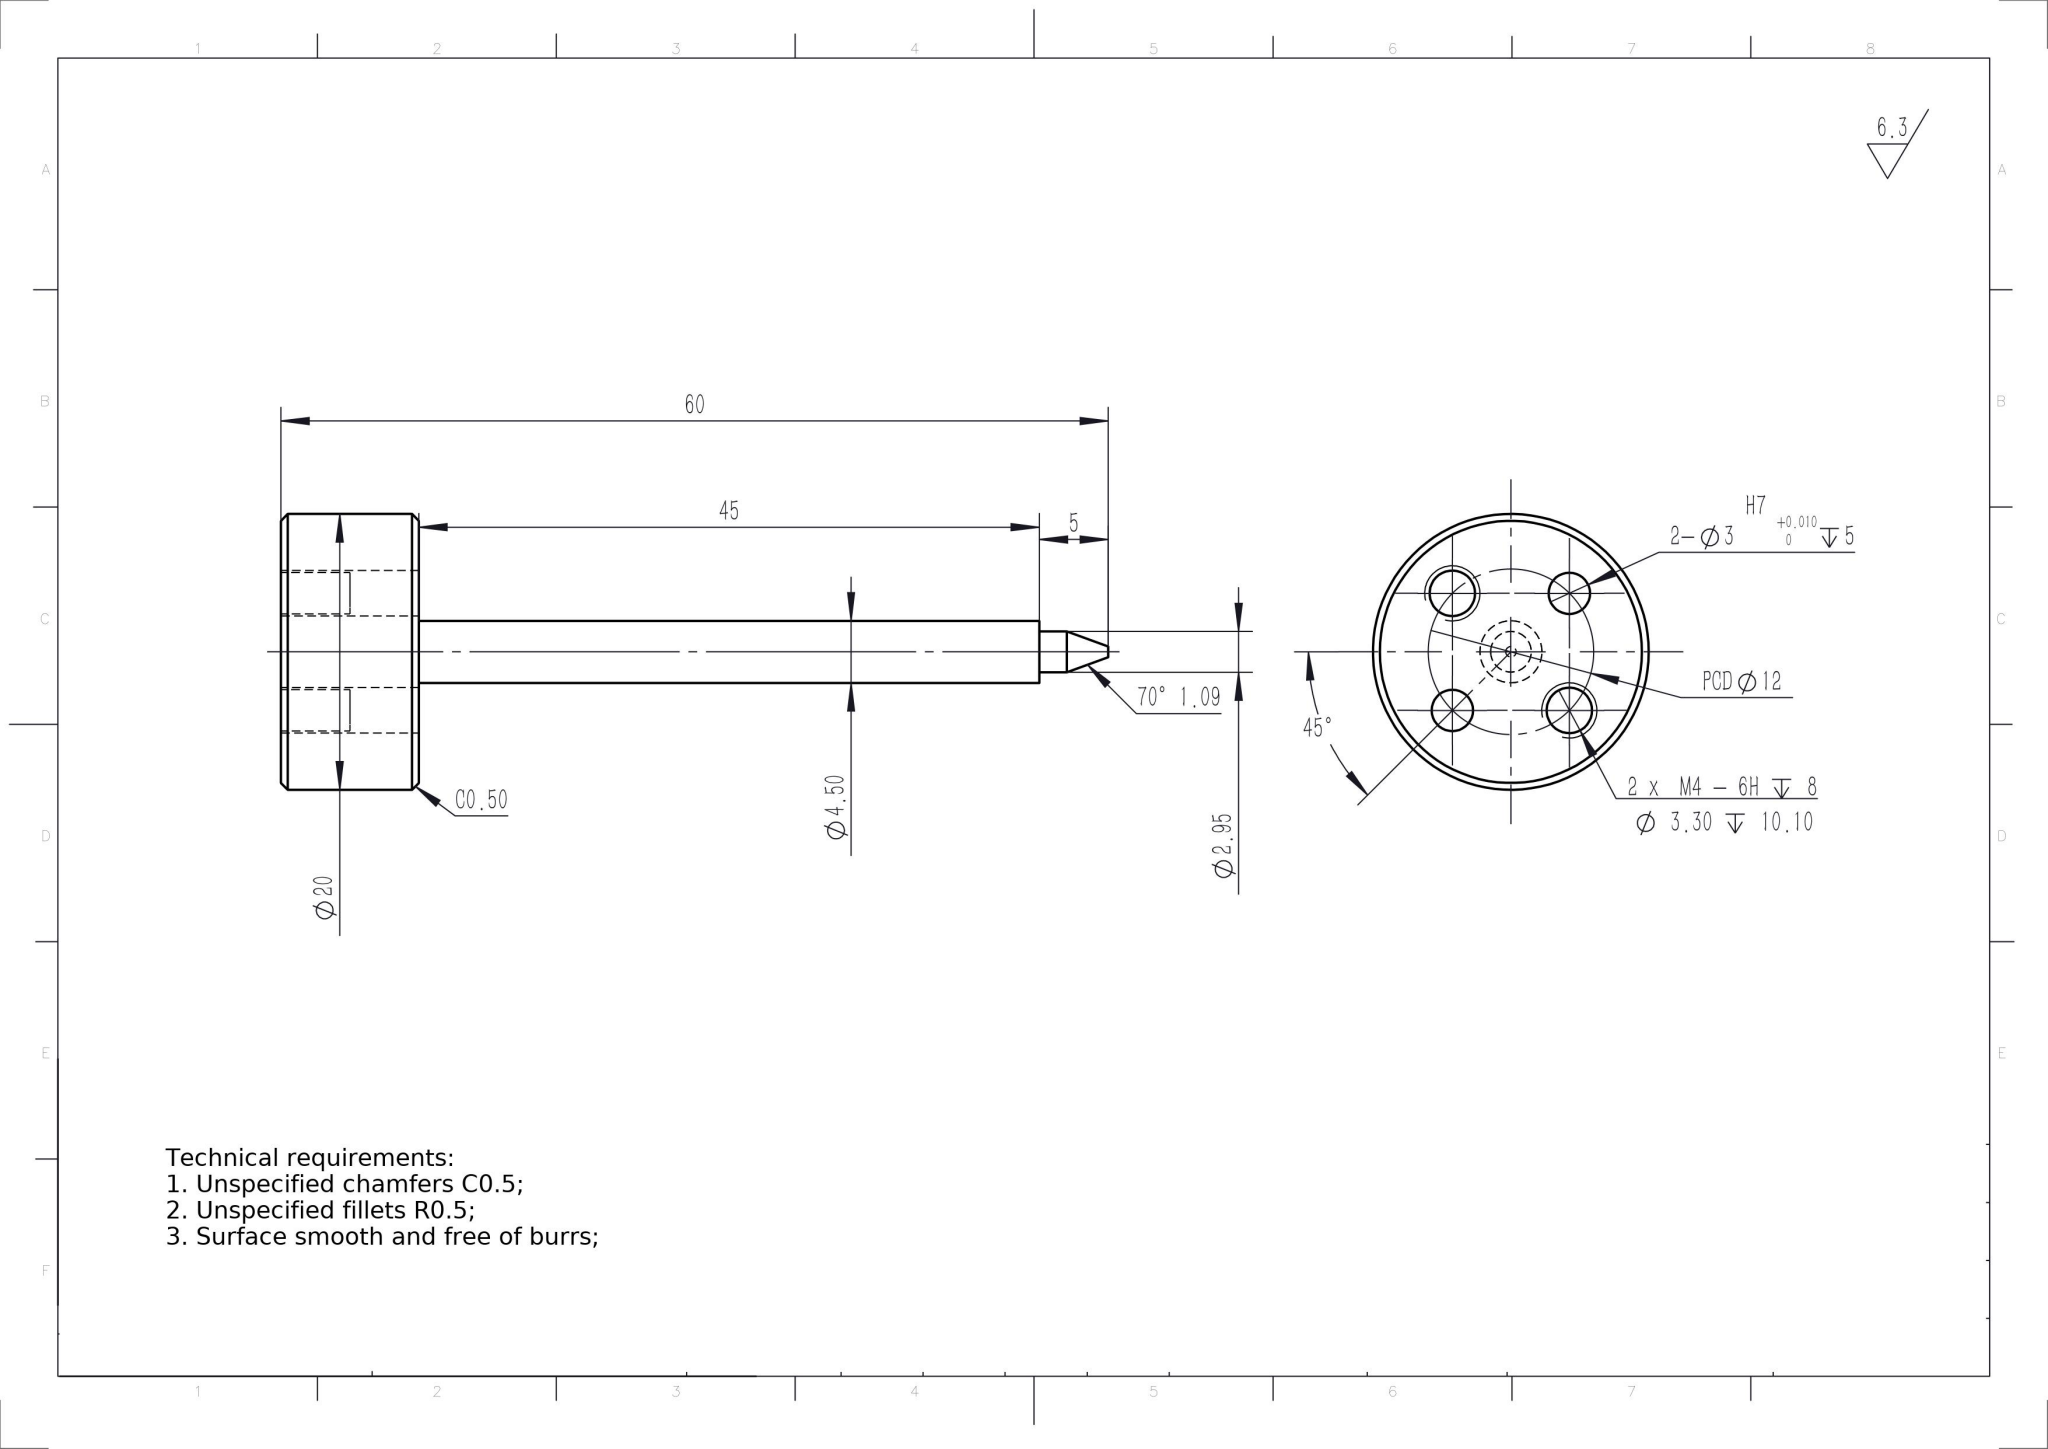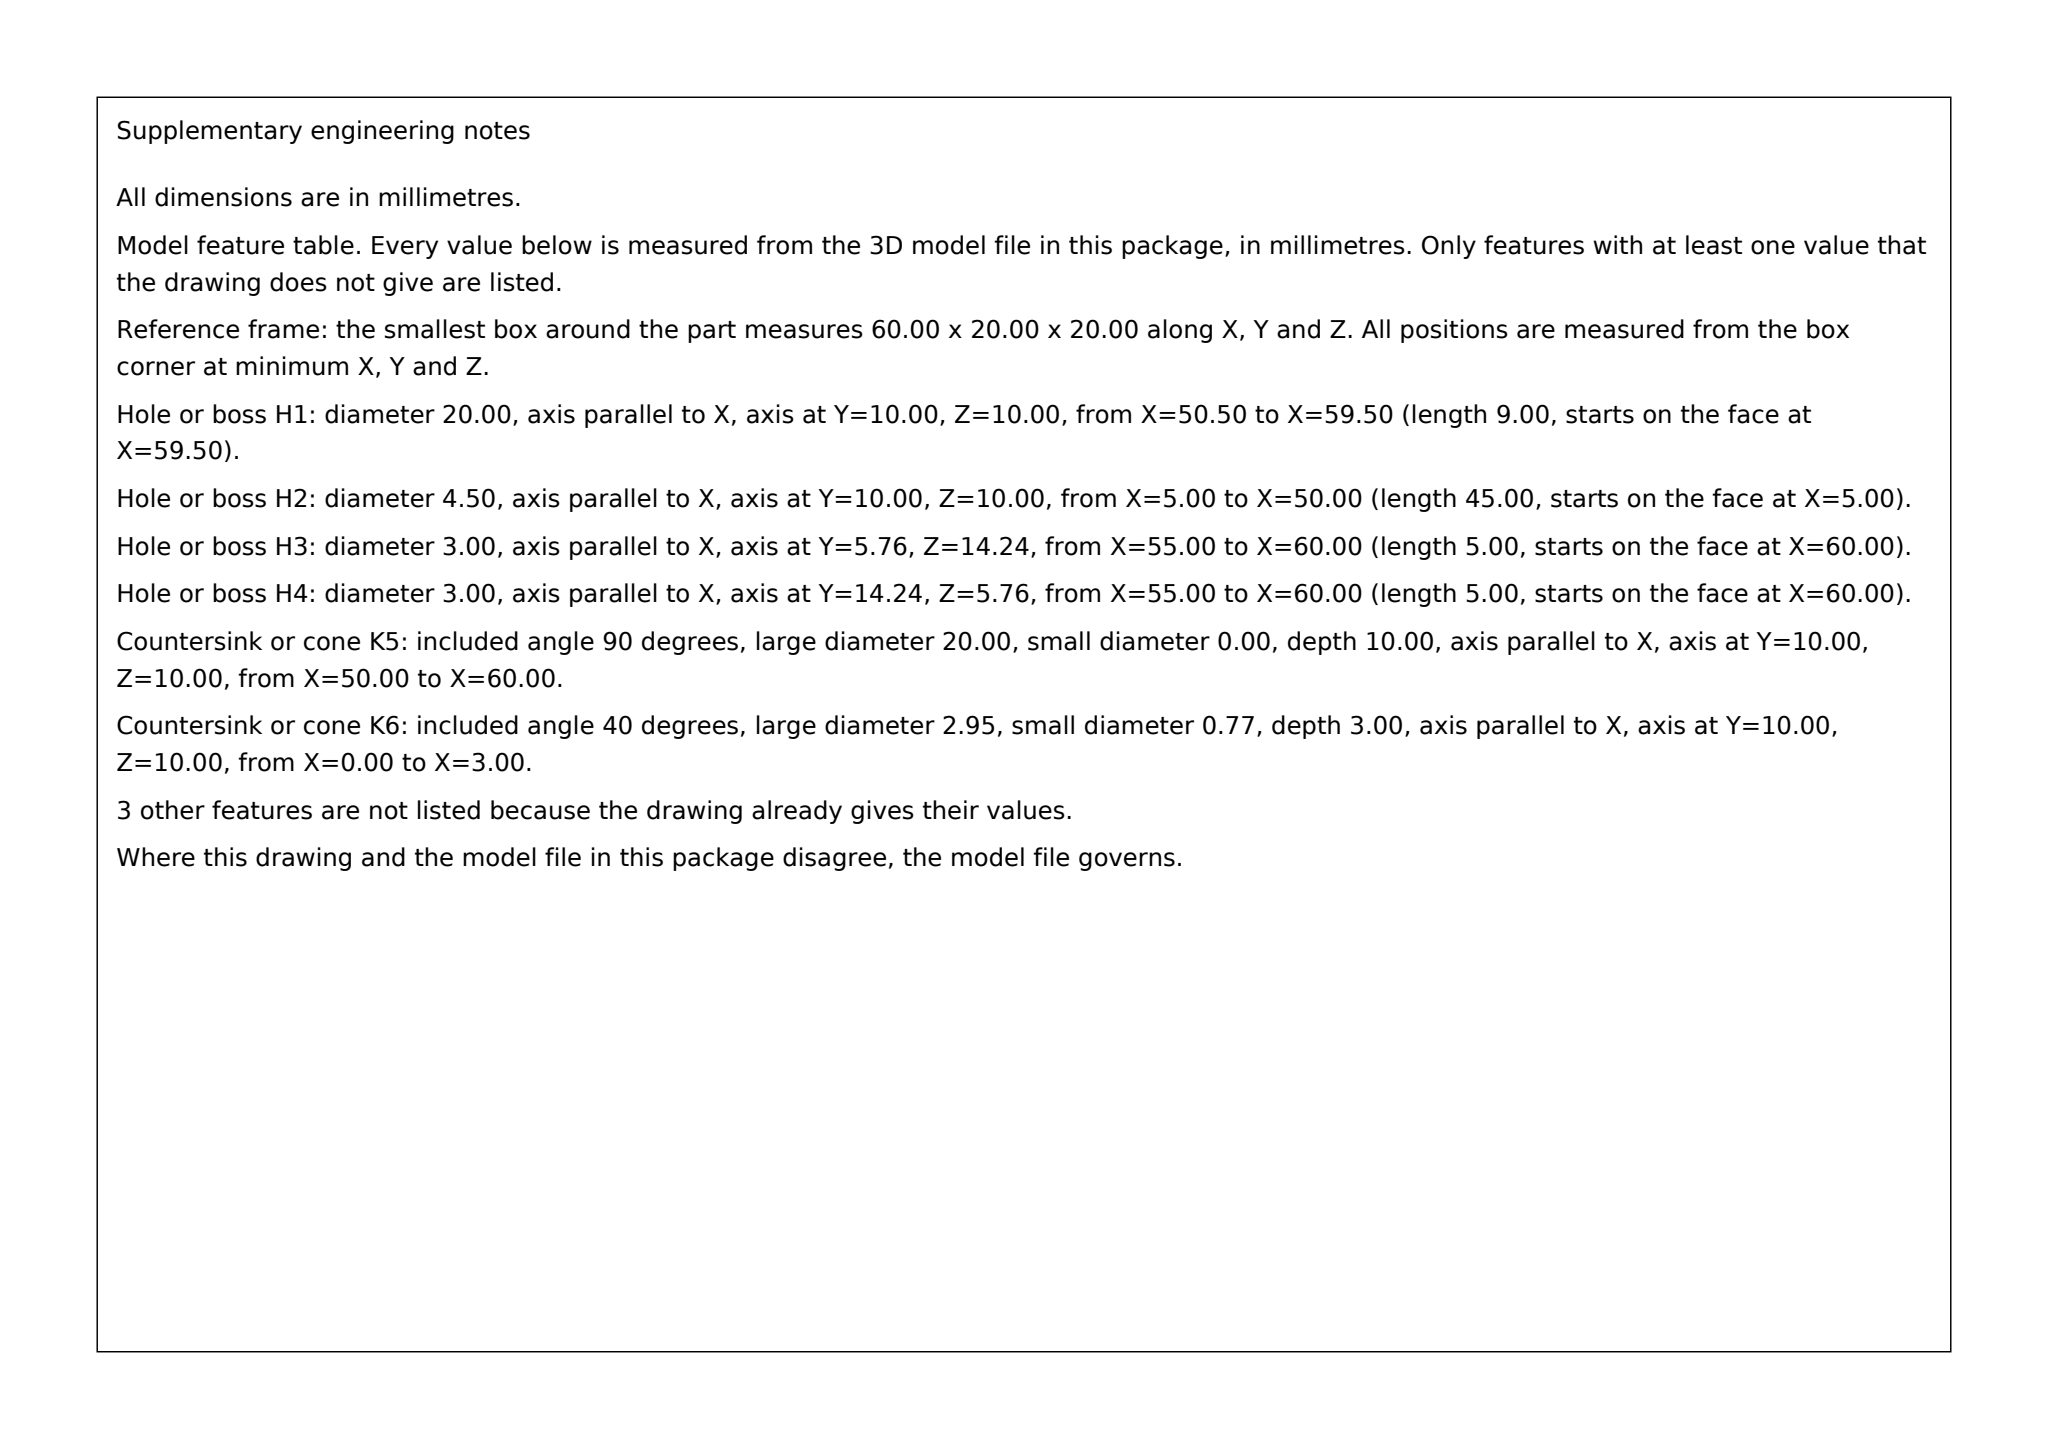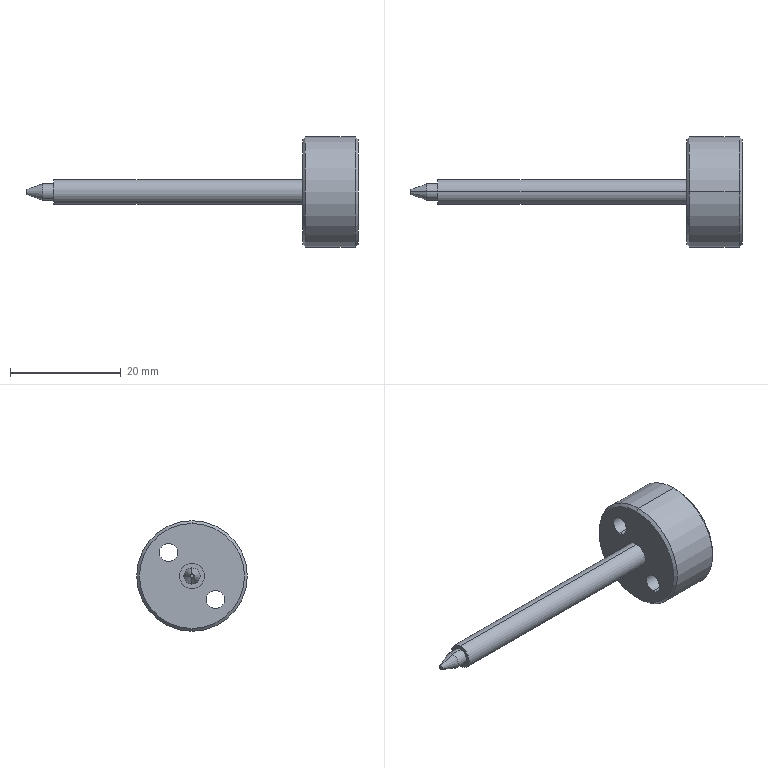Part | SolidWorks | mm | 1 solid | 26 faces | box 60 x 20 x 20 mm | volume 3623 mm3 | cylinder 14 | cone 6 | plane 6 | commonest cylinder face diameters 3.3 x4 3 x4 2.95 x2 20 x2 4.5 x2
build123d program:
from build123d import *

# Parameters (mm, degrees)
SKETCH1_R             = 2.25
BOSS_EXTRUDE1_DEPTH   = 45
SKETCH4_R             = 10
BOSS_EXTRUDE2_DEPTH   = 10
SKETCH6_R             = 2.5
CUT_EXTRUDE4_DEPTH    = 5
CHAMFER2_SIZE         = 0.5
SKETCH9_R             = 1.5
CUT_EXTRUDE5_DEPTH    = 5
M4_TAPPED_HOLE1_D     = 3.3
M4_TAPPED_HOLE1_DEPTH = 10.1
M4_TAPPED_HOLE1_TIP   = 0.9914
SKETCH15_R            = 1.475
BOSS_EXTRUDE3_DEPTH   = 5
BOSS_EXTRUDE4_START   = 5
SKETCH16_R            = 2.5
BOSS_EXTRUDE4_DEPTH   = 5
CHAMFER3_SIZE         = 3
CHAMFER3_SIZE2        = 1.092


with BuildPart() as part:
    # Sketch1 → Boss-Extrude1 (new body)
    with BuildSketch(Plane(origin=(0, 0, 0), x_dir=(0, 0, -1), z_dir=(1, 0, 0))):
        with Locations(Location((0, 0, 0), (0, 0, 180))):
            Circle(SKETCH1_R)
    extrude(amount=BOSS_EXTRUDE1_DEPTH)

    # Sketch4 → Boss-Extrude2 (add)
    with BuildSketch(Plane(origin=(45, 0, 0), x_dir=(0, 0, -1), z_dir=(1, 0, 0))):
        Circle(SKETCH4_R)
    extrude(amount=BOSS_EXTRUDE2_DEPTH)

    # Sketch6 → Cut-Extrude4 (cut)
    with BuildSketch(Plane(origin=(55, 0, 0), x_dir=(0, 0, -1), z_dir=(1, 0, 0))):
        Circle(SKETCH6_R)
    extrude(amount=-CUT_EXTRUDE4_DEPTH, mode=Mode.SUBTRACT)

    # Chamfer2
    chamfer2_edges = [part.edges().sort_by_distance(p)[0] for p in [
        (45, 0, 10),
        (55, 0, 10),
    ]]
    chamfer(chamfer2_edges, length=CHAMFER2_SIZE)

    # Sketch9 → Cut-Extrude5 (cut)
    with BuildSketch(Plane(origin=(55, 0, 0), x_dir=(0, 0, -1), z_dir=(1, 0, 0))):
        with Locations((4.243, 4.243)):
            Circle(SKETCH9_R)
        with Locations((-4.243, -4.243)):
            Circle(SKETCH9_R)
    extrude(amount=-CUT_EXTRUDE5_DEPTH, mode=Mode.SUBTRACT)

    # M4 Tapped Hole1
    with Locations(Plane(origin=(55, 0, 0), x_dir=(0, 0, -1), z_dir=(1, 0, 0))):
        with Locations((-4.243, 4.243), (4.243, -4.243)):
            Hole(M4_TAPPED_HOLE1_D / 2, depth=M4_TAPPED_HOLE1_DEPTH)
            with Locations((0, 0, -(M4_TAPPED_HOLE1_DEPTH + M4_TAPPED_HOLE1_TIP / 2))):  # 118° drill point
                Cone(0, M4_TAPPED_HOLE1_D / 2, M4_TAPPED_HOLE1_TIP, mode=Mode.SUBTRACT)

    # Sketch15 → Boss-Extrude3 (add)
    with BuildSketch(Plane.ZY):
        Circle(SKETCH15_R)
    extrude(amount=BOSS_EXTRUDE3_DEPTH)

    # Sketch16 → Boss-Extrude4 (add)
    with BuildSketch(Plane(origin=(50, 0, 0), x_dir=(0, 0, -1), z_dir=(1, 0, 0)).offset(BOSS_EXTRUDE4_START)):
        Circle(SKETCH16_R)
    extrude(amount=-BOSS_EXTRUDE4_DEPTH)

    # Chamfer3
    chamfer3_edges = [part.edges().sort_by_distance(p)[0] for p in [
        (-5, 0, -1.475),
    ]]
    chamfer3_side = [part.faces().sort_by_distance(p)[0] for p in [
        (-2.5, 0, -1.475),
    ]]
    chamfer(chamfer3_edges, length=CHAMFER3_SIZE, length2=CHAMFER3_SIZE2, reference=chamfer3_side[0])


solid = part.part
STEP:
#1=CARTESIAN_POINT('',(-5.,0.,0.3831));
#2=VERTEX_POINT('',#1);
#3=CARTESIAN_POINT('',(-5.,0.,-0.3831));
#4=VERTEX_POINT('',#3);
#5=CARTESIAN_POINT('',(-5.,0.,0.));
#6=DIRECTION('',(-1.,0.,0.));
#7=DIRECTION('',(0.,0.,1.));
#8=AXIS2_PLACEMENT_3D('',#5,#6,#7);
#9=CIRCLE('',#8,0.3831);
#10=EDGE_CURVE('',#2,#4,#9,.T.);
#11=ORIENTED_EDGE('',*,*,#10,.F.);
#12=CARTESIAN_POINT('',(-2.,0.,1.475));
#13=VERTEX_POINT('',#12);
#14=CARTESIAN_POINT('',(-5.,0.,0.3831));
#15=DIRECTION('',(0.9397,0.,0.342));
#16=VECTOR('',#15,1000.);
#17=LINE('',#14,#16);
#18=EDGE_CURVE('',#2,#13,#17,.T.);
#19=ORIENTED_EDGE('',*,*,#18,.T.);
#20=CARTESIAN_POINT('',(-2.,0.,-1.475));
#21=VERTEX_POINT('',#20);
#22=CARTESIAN_POINT('',(-2.,0.,0.));
#23=DIRECTION('',(1.,0.,0.));
#24=DIRECTION('',(0.,0.,1.));
#25=AXIS2_PLACEMENT_3D('',#22,#23,#24);
#26=CIRCLE('',#25,1.475);
#27=EDGE_CURVE('',#21,#13,#26,.T.);
#28=ORIENTED_EDGE('',*,*,#27,.F.);
#29=CARTESIAN_POINT('',(-5.,0.,-0.3831));
#30=DIRECTION('',(0.9397,0.,-0.342));
#31=VECTOR('',#30,1000.);
#32=LINE('',#29,#31);
#33=EDGE_CURVE('',#4,#21,#32,.T.);
#34=ORIENTED_EDGE('',*,*,#33,.F.);
#35=EDGE_LOOP('',(#11,#19,#28,#34));
#36=FACE_OUTER_BOUND('',#35,.T.);
#37=CARTESIAN_POINT('',(-5.,0.,0.));
#38=DIRECTION('',(1.,0.,0.));
#39=DIRECTION('',(0.,0.,-1.));
#40=AXIS2_PLACEMENT_3D('',#37,#38,#39);
#41=CONICAL_SURFACE('',#40,0.3831,0.3491);
#42=ADVANCED_FACE('',(#36),#41,.T.);
#43=ORIENTED_EDGE('',*,*,#27,.T.);
#44=CARTESIAN_POINT('',(0.,0.,1.475));
#45=VERTEX_POINT('',#44);
#46=CARTESIAN_POINT('',(-5.,0.,1.475));
#47=DIRECTION('',(1.,0.,0.));
#48=VECTOR('',#47,1000.);
#49=LINE('',#46,#48);
#50=EDGE_CURVE('',#13,#45,#49,.T.);
#51=ORIENTED_EDGE('',*,*,#50,.T.);
#52=CARTESIAN_POINT('',(0.,0.,-1.475));
#53=VERTEX_POINT('',#52);
#54=CARTESIAN_POINT('',(0.,0.,0.));
#55=DIRECTION('',(-1.,0.,0.));
#56=DIRECTION('',(0.,0.,1.));
#57=AXIS2_PLACEMENT_3D('',#54,#55,#56);
#58=CIRCLE('',#57,1.475);
#59=EDGE_CURVE('',#45,#53,#58,.T.);
#60=ORIENTED_EDGE('',*,*,#59,.T.);
#61=CARTESIAN_POINT('',(-5.,0.,-1.475));
#62=DIRECTION('',(1.,0.,0.));
#63=VECTOR('',#62,1000.);
#64=LINE('',#61,#63);
#65=EDGE_CURVE('',#21,#53,#64,.T.);
#66=ORIENTED_EDGE('',*,*,#65,.F.);
#67=EDGE_LOOP('',(#43,#51,#60,#66));
#68=FACE_OUTER_BOUND('',#67,.T.);
#69=CARTESIAN_POINT('',(-5.,0.,0.));
#70=DIRECTION('',(1.,0.,0.));
#71=DIRECTION('',(0.,0.,-1.));
#72=AXIS2_PLACEMENT_3D('',#69,#70,#71);
#73=CYLINDRICAL_SURFACE('',#72,1.475);
#74=ADVANCED_FACE('',(#68),#73,.T.);
#75=CARTESIAN_POINT('',(45.,4.243,5.893));
#76=VERTEX_POINT('',#75);
#77=CARTESIAN_POINT('',(45.,4.243,2.593));
#78=VERTEX_POINT('',#77);
#79=CARTESIAN_POINT('',(45.,4.243,4.243));
#80=DIRECTION('',(1.,0.,0.));
#81=DIRECTION('',(0.,0.,-1.));
#82=AXIS2_PLACEMENT_3D('',#79,#80,#81);
#83=CIRCLE('',#82,1.65);
#84=EDGE_CURVE('',#76,#78,#83,.T.);
#85=ORIENTED_EDGE('',*,*,#84,.F.);
#86=CARTESIAN_POINT('',(55.,4.243,5.893));
#87=VERTEX_POINT('',#86);
#88=CARTESIAN_POINT('',(55.,4.243,5.893));
#89=DIRECTION('',(1.,0.,0.));
#90=VECTOR('',#89,1000.);
#91=LINE('',#88,#90);
#92=EDGE_CURVE('',#76,#87,#91,.T.);
#93=ORIENTED_EDGE('',*,*,#92,.T.);
#94=CARTESIAN_POINT('',(55.,4.243,2.593));
#95=VERTEX_POINT('',#94);
#96=CARTESIAN_POINT('',(55.,4.243,4.243));
#97=DIRECTION('',(1.,0.,0.));
#98=DIRECTION('',(0.,0.,-1.));
#99=AXIS2_PLACEMENT_3D('',#96,#97,#98);
#100=CIRCLE('',#99,1.65);
#101=EDGE_CURVE('',#87,#95,#100,.T.);
#102=ORIENTED_EDGE('',*,*,#101,.T.);
#103=CARTESIAN_POINT('',(55.,4.243,2.593));
#104=DIRECTION('',(1.,0.,0.));
#105=VECTOR('',#104,1000.);
#106=LINE('',#103,#105);
#107=EDGE_CURVE('',#78,#95,#106,.T.);
#108=ORIENTED_EDGE('',*,*,#107,.F.);
#109=EDGE_LOOP('',(#85,#93,#102,#108));
#110=FACE_OUTER_BOUND('',#109,.T.);
#111=CARTESIAN_POINT('',(55.,4.243,4.243));
#112=DIRECTION('',(1.,0.,0.));
#113=DIRECTION('',(0.,0.,-1.));
#114=AXIS2_PLACEMENT_3D('',#111,#112,#113);
#115=CYLINDRICAL_SURFACE('',#114,1.65);
#116=ADVANCED_FACE('',(#110),#115,.F.);
#117=CARTESIAN_POINT('',(45.,-4.243,-2.593));
#118=VERTEX_POINT('',#117);
#119=CARTESIAN_POINT('',(45.,-4.243,-5.893));
#120=VERTEX_POINT('',#119);
#121=CARTESIAN_POINT('',(45.,-4.243,-4.243));
#122=DIRECTION('',(1.,0.,0.));
#123=DIRECTION('',(0.,0.,-1.));
#124=AXIS2_PLACEMENT_3D('',#121,#122,#123);
#125=CIRCLE('',#124,1.65);
#126=EDGE_CURVE('',#118,#120,#125,.T.);
#127=ORIENTED_EDGE('',*,*,#126,.F.);
#128=CARTESIAN_POINT('',(55.,-4.243,-2.593));
#129=VERTEX_POINT('',#128);
#130=CARTESIAN_POINT('',(55.,-4.243,-2.593));
#131=DIRECTION('',(1.,0.,0.));
#132=VECTOR('',#131,1000.);
#133=LINE('',#130,#132);
#134=EDGE_CURVE('',#118,#129,#133,.T.);
#135=ORIENTED_EDGE('',*,*,#134,.T.);
#136=CARTESIAN_POINT('',(55.,-4.243,-5.893));
#137=VERTEX_POINT('',#136);
#138=CARTESIAN_POINT('',(55.,-4.243,-4.243));
#139=DIRECTION('',(1.,0.,0.));
#140=DIRECTION('',(0.,0.,-1.));
#141=AXIS2_PLACEMENT_3D('',#138,#139,#140);
#142=CIRCLE('',#141,1.65);
#143=EDGE_CURVE('',#129,#137,#142,.T.);
#144=ORIENTED_EDGE('',*,*,#143,.T.);
#145=CARTESIAN_POINT('',(55.,-4.243,-5.893));
#146=DIRECTION('',(1.,0.,0.));
#147=VECTOR('',#146,1000.);
#148=LINE('',#145,#147);
#149=EDGE_CURVE('',#120,#137,#148,.T.);
#150=ORIENTED_EDGE('',*,*,#149,.F.);
#151=EDGE_LOOP('',(#127,#135,#144,#150));
#152=FACE_OUTER_BOUND('',#151,.T.);
#153=CARTESIAN_POINT('',(55.,-4.243,-4.243));
#154=DIRECTION('',(1.,0.,0.));
#155=DIRECTION('',(0.,0.,-1.));
#156=AXIS2_PLACEMENT_3D('',#153,#154,#155);
#157=CYLINDRICAL_SURFACE('',#156,1.65);
#158=ADVANCED_FACE('',(#152),#157,.F.);
#159=CARTESIAN_POINT('',(50.,4.243,-2.743));
#160=VERTEX_POINT('',#159);
#161=CARTESIAN_POINT('',(50.,4.243,-5.743));
#162=VERTEX_POINT('',#161);
#163=CARTESIAN_POINT('',(50.,4.243,-4.243));
#164=DIRECTION('',(1.,0.,0.));
#165=DIRECTION('',(0.,0.,-1.));
#166=AXIS2_PLACEMENT_3D('',#163,#164,#165);
#167=CIRCLE('',#166,1.5);
#168=EDGE_CURVE('',#160,#162,#167,.T.);
#169=ORIENTED_EDGE('',*,*,#168,.F.);
#170=CARTESIAN_POINT('',(55.,4.243,-2.743));
#171=VERTEX_POINT('',#170);
#172=CARTESIAN_POINT('',(50.,4.243,-2.743));
#173=DIRECTION('',(1.,0.,0.));
#174=VECTOR('',#173,1000.);
#175=LINE('',#172,#174);
#176=EDGE_CURVE('',#160,#171,#175,.T.);
#177=ORIENTED_EDGE('',*,*,#176,.T.);
#178=CARTESIAN_POINT('',(55.,4.243,-5.743));
#179=VERTEX_POINT('',#178);
#180=CARTESIAN_POINT('',(55.,4.243,-4.243));
#181=DIRECTION('',(1.,0.,0.));
#182=DIRECTION('',(0.,0.,-1.));
#183=AXIS2_PLACEMENT_3D('',#180,#181,#182);
#184=CIRCLE('',#183,1.5);
#185=EDGE_CURVE('',#171,#179,#184,.T.);
#186=ORIENTED_EDGE('',*,*,#185,.T.);
#187=CARTESIAN_POINT('',(50.,4.243,-5.743));
#188=DIRECTION('',(1.,0.,0.));
#189=VECTOR('',#188,1000.);
#190=LINE('',#187,#189);
#191=EDGE_CURVE('',#162,#179,#190,.T.);
#192=ORIENTED_EDGE('',*,*,#191,.F.);
#193=EDGE_LOOP('',(#169,#177,#186,#192));
#194=FACE_OUTER_BOUND('',#193,.T.);
#195=CARTESIAN_POINT('',(50.,4.243,-4.243));
#196=DIRECTION('',(1.,0.,0.));
#197=DIRECTION('',(0.,0.,-1.));
#198=AXIS2_PLACEMENT_3D('',#195,#196,#197);
#199=CYLINDRICAL_SURFACE('',#198,1.5);
#200=ADVANCED_FACE('',(#194),#199,.F.);
#201=CARTESIAN_POINT('',(50.,-4.243,5.743));
#202=VERTEX_POINT('',#201);
#203=CARTESIAN_POINT('',(50.,-4.243,2.743));
#204=VERTEX_POINT('',#203);
#205=CARTESIAN_POINT('',(50.,-4.243,4.243));
#206=DIRECTION('',(1.,0.,0.));
#207=DIRECTION('',(0.,0.,-1.));
#208=AXIS2_PLACEMENT_3D('',#205,#206,#207);
#209=CIRCLE('',#208,1.5);
#210=EDGE_CURVE('',#202,#204,#209,.T.);
#211=ORIENTED_EDGE('',*,*,#210,.F.);
#212=CARTESIAN_POINT('',(55.,-4.243,5.743));
#213=VERTEX_POINT('',#212);
#214=CARTESIAN_POINT('',(50.,-4.243,5.743));
#215=DIRECTION('',(1.,0.,0.));
#216=VECTOR('',#215,1000.);
#217=LINE('',#214,#216);
#218=EDGE_CURVE('',#202,#213,#217,.T.);
#219=ORIENTED_EDGE('',*,*,#218,.T.);
#220=CARTESIAN_POINT('',(55.,-4.243,2.743));
#221=VERTEX_POINT('',#220);
#222=CARTESIAN_POINT('',(55.,-4.243,4.243));
#223=DIRECTION('',(1.,0.,0.));
#224=DIRECTION('',(0.,0.,-1.));
#225=AXIS2_PLACEMENT_3D('',#222,#223,#224);
#226=CIRCLE('',#225,1.5);
#227=EDGE_CURVE('',#213,#221,#226,.T.);
#228=ORIENTED_EDGE('',*,*,#227,.T.);
#229=CARTESIAN_POINT('',(50.,-4.243,2.743));
#230=DIRECTION('',(1.,0.,0.));
#231=VECTOR('',#230,1000.);
#232=LINE('',#229,#231);
#233=EDGE_CURVE('',#204,#221,#232,.T.);
#234=ORIENTED_EDGE('',*,*,#233,.F.);
#235=EDGE_LOOP('',(#211,#219,#228,#234));
#236=FACE_OUTER_BOUND('',#235,.T.);
#237=CARTESIAN_POINT('',(50.,-4.243,4.243));
#238=DIRECTION('',(1.,0.,0.));
#239=DIRECTION('',(0.,0.,-1.));
#240=AXIS2_PLACEMENT_3D('',#237,#238,#239);
#241=CYLINDRICAL_SURFACE('',#240,1.5);
#242=ADVANCED_FACE('',(#236),#241,.F.);
#243=CARTESIAN_POINT('',(45.,0.,9.5));
#244=VERTEX_POINT('',#243);
#245=CARTESIAN_POINT('',(45.,0.,-9.5));
#246=VERTEX_POINT('',#245);
#247=CARTESIAN_POINT('',(45.,0.,0.));
#248=DIRECTION('',(-1.,0.,0.));
#249=DIRECTION('',(0.,0.,-1.));
#250=AXIS2_PLACEMENT_3D('',#247,#248,#249);
#251=CIRCLE('',#250,9.5);
#252=EDGE_CURVE('',#244,#246,#251,.T.);
#253=ORIENTED_EDGE('',*,*,#252,.F.);
#254=CARTESIAN_POINT('',(45.5,0.,10.));
#255=VERTEX_POINT('',#254);
#256=CARTESIAN_POINT('',(45.5,0.,10.));
#257=DIRECTION('',(0.7071,0.,0.7071));
#258=VECTOR('',#257,1000.);
#259=LINE('',#256,#258);
#260=EDGE_CURVE('',#244,#255,#259,.T.);
#261=ORIENTED_EDGE('',*,*,#260,.T.);
#262=CARTESIAN_POINT('',(45.5,0.,-10.));
#263=VERTEX_POINT('',#262);
#264=CARTESIAN_POINT('',(45.5,0.,0.));
#265=DIRECTION('',(1.,0.,0.));
#266=DIRECTION('',(0.,0.,-1.));
#267=AXIS2_PLACEMENT_3D('',#264,#265,#266);
#268=CIRCLE('',#267,10.);
#269=EDGE_CURVE('',#263,#255,#268,.T.);
#270=ORIENTED_EDGE('',*,*,#269,.F.);
#271=CARTESIAN_POINT('',(45.5,0.,-10.));
#272=DIRECTION('',(0.7071,0.,-0.7071));
#273=VECTOR('',#272,1000.);
#274=LINE('',#271,#273);
#275=EDGE_CURVE('',#246,#263,#274,.T.);
#276=ORIENTED_EDGE('',*,*,#275,.F.);
#277=EDGE_LOOP('',(#253,#261,#270,#276));
#278=FACE_OUTER_BOUND('',#277,.T.);
#279=CARTESIAN_POINT('',(45.5,0.,0.));
#280=DIRECTION('',(1.,0.,0.));
#281=DIRECTION('',(0.,0.,-1.));
#282=AXIS2_PLACEMENT_3D('',#279,#280,#281);
#283=CONICAL_SURFACE('',#282,10.,0.7854);
#284=ADVANCED_FACE('',(#278),#283,.T.);
#285=CARTESIAN_POINT('',(55.,0.,-9.5));
#286=VERTEX_POINT('',#285);
#287=CARTESIAN_POINT('',(55.,0.,9.5));
#288=VERTEX_POINT('',#287);
#289=CARTESIAN_POINT('',(55.,0.,0.));
#290=DIRECTION('',(1.,0.,0.));
#291=DIRECTION('',(0.,0.,-1.));
#292=AXIS2_PLACEMENT_3D('',#289,#290,#291);
#293=CIRCLE('',#292,9.5);
#294=EDGE_CURVE('',#286,#288,#293,.T.);
#295=ORIENTED_EDGE('',*,*,#294,.F.);
#296=CARTESIAN_POINT('',(54.5,0.,-10.));
#297=VERTEX_POINT('',#296);
#298=CARTESIAN_POINT('',(55.,0.,-9.5));
#299=DIRECTION('',(-0.7071,0.,-0.7071));
#300=VECTOR('',#299,1000.);
#301=LINE('',#298,#300);
#302=EDGE_CURVE('',#286,#297,#301,.T.);
#303=ORIENTED_EDGE('',*,*,#302,.T.);
#304=CARTESIAN_POINT('',(54.5,0.,10.));
#305=VERTEX_POINT('',#304);
#306=CARTESIAN_POINT('',(54.5,0.,0.));
#307=DIRECTION('',(-1.,0.,0.));
#308=DIRECTION('',(0.,0.,-1.));
#309=AXIS2_PLACEMENT_3D('',#306,#307,#308);
#310=CIRCLE('',#309,10.);
#311=EDGE_CURVE('',#305,#297,#310,.T.);
#312=ORIENTED_EDGE('',*,*,#311,.F.);
#313=CARTESIAN_POINT('',(55.,0.,9.5));
#314=DIRECTION('',(-0.7071,0.,0.7071));
#315=VECTOR('',#314,1000.);
#316=LINE('',#313,#315);
#317=EDGE_CURVE('',#288,#305,#316,.T.);
#318=ORIENTED_EDGE('',*,*,#317,.F.);
#319=EDGE_LOOP('',(#295,#303,#312,#318));
#320=FACE_OUTER_BOUND('',#319,.T.);
#321=CARTESIAN_POINT('',(55.,0.,0.));
#322=DIRECTION('',(-1.,0.,0.));
#323=DIRECTION('',(0.,0.,1.));
#324=AXIS2_PLACEMENT_3D('',#321,#322,#323);
#325=CONICAL_SURFACE('',#324,9.5,0.7854);
#326=ADVANCED_FACE('',(#320),#325,.T.);
#327=ORIENTED_EDGE('',*,*,#311,.T.);
#328=CARTESIAN_POINT('',(55.,0.,-10.));
#329=DIRECTION('',(-1.,0.,0.));
#330=VECTOR('',#329,1000.);
#331=LINE('',#328,#330);
#332=EDGE_CURVE('',#297,#263,#331,.T.);
#333=ORIENTED_EDGE('',*,*,#332,.T.);
#334=ORIENTED_EDGE('',*,*,#269,.T.);
#335=CARTESIAN_POINT('',(55.,0.,10.));
#336=DIRECTION('',(-1.,0.,0.));
#337=VECTOR('',#336,1000.);
#338=LINE('',#335,#337);
#339=EDGE_CURVE('',#305,#255,#338,.T.);
#340=ORIENTED_EDGE('',*,*,#339,.F.);
#341=EDGE_LOOP('',(#327,#333,#334,#340));
#342=FACE_OUTER_BOUND('',#341,.T.);
#343=CARTESIAN_POINT('',(55.,0.,0.));
#344=DIRECTION('',(-1.,0.,0.));
#345=DIRECTION('',(0.,0.,1.));
#346=AXIS2_PLACEMENT_3D('',#343,#344,#345);
#347=CYLINDRICAL_SURFACE('',#346,10.);
#348=ADVANCED_FACE('',(#342),#347,.T.);
#349=CARTESIAN_POINT('',(45.,0.,-2.25));
#350=VERTEX_POINT('',#349);
#351=CARTESIAN_POINT('',(45.,0.,2.25));
#352=VERTEX_POINT('',#351);
#353=CARTESIAN_POINT('',(45.,0.,0.));
#354=DIRECTION('',(1.,0.,0.));
#355=DIRECTION('',(0.,0.,-1.));
#356=AXIS2_PLACEMENT_3D('',#353,#354,#355);
#357=CIRCLE('',#356,2.25);
#358=EDGE_CURVE('',#350,#352,#357,.T.);
#359=ORIENTED_EDGE('',*,*,#358,.F.);
#360=CARTESIAN_POINT('',(0.,0.,-2.25));
#361=VERTEX_POINT('',#360);
#362=CARTESIAN_POINT('',(45.,0.,-2.25));
#363=DIRECTION('',(-1.,0.,0.));
#364=VECTOR('',#363,1000.);
#365=LINE('',#362,#364);
#366=EDGE_CURVE('',#350,#361,#365,.T.);
#367=ORIENTED_EDGE('',*,*,#366,.T.);
#368=CARTESIAN_POINT('',(0.,0.,2.25));
#369=VERTEX_POINT('',#368);
#370=CARTESIAN_POINT('',(0.,0.,0.));
#371=DIRECTION('',(1.,0.,0.));
#372=DIRECTION('',(0.,0.,-1.));
#373=AXIS2_PLACEMENT_3D('',#370,#371,#372);
#374=CIRCLE('',#373,2.25);
#375=EDGE_CURVE('',#361,#369,#374,.T.);
#376=ORIENTED_EDGE('',*,*,#375,.T.);
#377=CARTESIAN_POINT('',(45.,0.,2.25));
#378=DIRECTION('',(-1.,0.,0.));
#379=VECTOR('',#378,1000.);
#380=LINE('',#377,#379);
#381=EDGE_CURVE('',#352,#369,#380,.T.);
#382=ORIENTED_EDGE('',*,*,#381,.F.);
#383=EDGE_LOOP('',(#359,#367,#376,#382));
#384=FACE_OUTER_BOUND('',#383,.T.);
#385=CARTESIAN_POINT('',(45.,0.,0.));
#386=DIRECTION('',(-1.,0.,0.));
#387=DIRECTION('',(0.,0.,1.));
#388=AXIS2_PLACEMENT_3D('',#385,#386,#387);
#389=CYLINDRICAL_SURFACE('',#388,2.25);
#390=ADVANCED_FACE('',(#384),#389,.T.);
#391=ORIENTED_EDGE('',*,*,#366,.F.);
#392=CARTESIAN_POINT('',(45.,0.,0.));
#393=DIRECTION('',(1.,0.,0.));
#394=DIRECTION('',(0.,0.,-1.));
#395=AXIS2_PLACEMENT_3D('',#392,#393,#394);
#396=CIRCLE('',#395,2.25);
#397=EDGE_CURVE('',#352,#350,#396,.T.);
#398=ORIENTED_EDGE('',*,*,#397,.F.);
#399=ORIENTED_EDGE('',*,*,#381,.T.);
#400=CARTESIAN_POINT('',(0.,0.,0.));
#401=DIRECTION('',(1.,0.,0.));
#402=DIRECTION('',(0.,0.,-1.));
#403=AXIS2_PLACEMENT_3D('',#400,#401,#402);
#404=CIRCLE('',#403,2.25);
#405=EDGE_CURVE('',#369,#361,#404,.T.);
#406=ORIENTED_EDGE('',*,*,#405,.T.);
#407=EDGE_LOOP('',(#391,#398,#399,#406));
#408=FACE_OUTER_BOUND('',#407,.T.);
#409=CARTESIAN_POINT('',(45.,0.,0.));
#410=DIRECTION('',(-1.,0.,0.));
#411=DIRECTION('',(0.,0.,1.));
#412=AXIS2_PLACEMENT_3D('',#409,#410,#411);
#413=CYLINDRICAL_SURFACE('',#412,2.25);
#414=ADVANCED_FACE('',(#408),#413,.T.);
#415=CARTESIAN_POINT('',(0.,0.,0.));
#416=DIRECTION('',(-1.,0.,0.));
#417=DIRECTION('',(0.,0.,1.));
#418=AXIS2_PLACEMENT_3D('',#415,#416,#417);
#419=CIRCLE('',#418,1.475);
#420=EDGE_CURVE('',#53,#45,#419,.T.);
#421=ORIENTED_EDGE('',*,*,#420,.F.);
#422=ORIENTED_EDGE('',*,*,#59,.F.);
#423=EDGE_LOOP('',(#421,#422));
#424=FACE_BOUND('',#423,.T.);
#425=ORIENTED_EDGE('',*,*,#405,.F.);
#426=ORIENTED_EDGE('',*,*,#375,.F.);
#427=EDGE_LOOP('',(#425,#426));
#428=FACE_OUTER_BOUND('',#427,.T.);
#429=CARTESIAN_POINT('',(0.,0.,0.));
#430=DIRECTION('',(1.,0.,0.));
#431=DIRECTION('',(0.,0.,-1.));
#432=AXIS2_PLACEMENT_3D('',#429,#430,#431);
#433=PLANE('',#432);
#434=ADVANCED_FACE('',(#424,#428),#433,.F.);
#435=ORIENTED_EDGE('',*,*,#332,.F.);
#436=CARTESIAN_POINT('',(54.5,0.,0.));
#437=DIRECTION('',(-1.,0.,0.));
#438=DIRECTION('',(0.,0.,-1.));
#439=AXIS2_PLACEMENT_3D('',#436,#437,#438);
#440=CIRCLE('',#439,10.);
#441=EDGE_CURVE('',#297,#305,#440,.T.);
#442=ORIENTED_EDGE('',*,*,#441,.T.);
#443=ORIENTED_EDGE('',*,*,#339,.T.);
#444=CARTESIAN_POINT('',(45.5,0.,0.));
#445=DIRECTION('',(1.,0.,0.));
#446=DIRECTION('',(0.,0.,-1.));
#447=AXIS2_PLACEMENT_3D('',#444,#445,#446);
#448=CIRCLE('',#447,10.);
#449=EDGE_CURVE('',#255,#263,#448,.T.);
#450=ORIENTED_EDGE('',*,*,#449,.T.);
#451=EDGE_LOOP('',(#435,#442,#443,#450));
#452=FACE_OUTER_BOUND('',#451,.T.);
#453=CARTESIAN_POINT('',(55.,0.,0.));
#454=DIRECTION('',(-1.,0.,0.));
#455=DIRECTION('',(0.,0.,1.));
#456=AXIS2_PLACEMENT_3D('',#453,#454,#455);
#457=CYLINDRICAL_SURFACE('',#456,10.);
#458=ADVANCED_FACE('',(#452),#457,.T.);
#459=CARTESIAN_POINT('',(55.,4.243,4.243));
#460=DIRECTION('',(1.,0.,0.));
#461=DIRECTION('',(0.,0.,-1.));
#462=AXIS2_PLACEMENT_3D('',#459,#460,#461);
#463=CIRCLE('',#462,1.65);
#464=EDGE_CURVE('',#95,#87,#463,.T.);
#465=ORIENTED_EDGE('',*,*,#464,.F.);
#466=ORIENTED_EDGE('',*,*,#101,.F.);
#467=EDGE_LOOP('',(#465,#466));
#468=FACE_BOUND('',#467,.T.);
#469=CARTESIAN_POINT('',(55.,-4.243,-4.243));
#470=DIRECTION('',(1.,0.,0.));
#471=DIRECTION('',(0.,0.,-1.));
#472=AXIS2_PLACEMENT_3D('',#469,#470,#471);
#473=CIRCLE('',#472,1.65);
#474=EDGE_CURVE('',#137,#129,#473,.T.);
#475=ORIENTED_EDGE('',*,*,#474,.F.);
#476=ORIENTED_EDGE('',*,*,#143,.F.);
#477=EDGE_LOOP('',(#475,#476));
#478=FACE_BOUND('',#477,.T.);
#479=CARTESIAN_POINT('',(55.,4.243,-4.243));
#480=DIRECTION('',(1.,0.,0.));
#481=DIRECTION('',(0.,0.,-1.));
#482=AXIS2_PLACEMENT_3D('',#479,#480,#481);
#483=CIRCLE('',#482,1.5);
#484=EDGE_CURVE('',#179,#171,#483,.T.);
#485=ORIENTED_EDGE('',*,*,#484,.F.);
#486=ORIENTED_EDGE('',*,*,#185,.F.);
#487=EDGE_LOOP('',(#485,#486));
#488=FACE_BOUND('',#487,.T.);
#489=CARTESIAN_POINT('',(55.,-4.243,4.243));
#490=DIRECTION('',(1.,0.,0.));
#491=DIRECTION('',(0.,0.,-1.));
#492=AXIS2_PLACEMENT_3D('',#489,#490,#491);
#493=CIRCLE('',#492,1.5);
#494=EDGE_CURVE('',#221,#213,#493,.T.);
#495=ORIENTED_EDGE('',*,*,#494,.F.);
#496=ORIENTED_EDGE('',*,*,#227,.F.);
#497=EDGE_LOOP('',(#495,#496));
#498=FACE_BOUND('',#497,.T.);
#499=CARTESIAN_POINT('',(55.,0.,0.));
#500=DIRECTION('',(1.,0.,0.));
#501=DIRECTION('',(0.,0.,-1.));
#502=AXIS2_PLACEMENT_3D('',#499,#500,#501);
#503=CIRCLE('',#502,9.5);
#504=EDGE_CURVE('',#288,#286,#503,.T.);
#505=ORIENTED_EDGE('',*,*,#504,.T.);
#506=ORIENTED_EDGE('',*,*,#294,.T.);
#507=EDGE_LOOP('',(#505,#506));
#508=FACE_OUTER_BOUND('',#507,.T.);
#509=CARTESIAN_POINT('',(55.,0.,0.));
#510=DIRECTION('',(1.,0.,0.));
#511=DIRECTION('',(0.,0.,-1.));
#512=AXIS2_PLACEMENT_3D('',#509,#510,#511);
#513=PLANE('',#512);
#514=ADVANCED_FACE('',(#468,#478,#488,#498,#508),#513,.T.);
#515=CARTESIAN_POINT('',(45.,4.243,4.243));
#516=DIRECTION('',(1.,0.,0.));
#517=DIRECTION('',(0.,0.,-1.));
#518=AXIS2_PLACEMENT_3D('',#515,#516,#517);
#519=CIRCLE('',#518,1.65);
#520=EDGE_CURVE('',#78,#76,#519,.T.);
#521=ORIENTED_EDGE('',*,*,#520,.T.);
#522=ORIENTED_EDGE('',*,*,#84,.T.);
#523=EDGE_LOOP('',(#521,#522));
#524=FACE_BOUND('',#523,.T.);
#525=CARTESIAN_POINT('',(45.,-4.243,-4.243));
#526=DIRECTION('',(1.,0.,0.));
#527=DIRECTION('',(0.,0.,-1.));
#528=AXIS2_PLACEMENT_3D('',#525,#526,#527);
#529=CIRCLE('',#528,1.65);
#530=EDGE_CURVE('',#120,#118,#529,.T.);
#531=ORIENTED_EDGE('',*,*,#530,.T.);
#532=ORIENTED_EDGE('',*,*,#126,.T.);
#533=EDGE_LOOP('',(#531,#532));
#534=FACE_BOUND('',#533,.T.);
#535=CARTESIAN_POINT('',(45.,0.,0.));
#536=DIRECTION('',(-1.,0.,0.));
#537=DIRECTION('',(0.,0.,-1.));
#538=AXIS2_PLACEMENT_3D('',#535,#536,#537);
#539=CIRCLE('',#538,9.5);
#540=EDGE_CURVE('',#246,#244,#539,.T.);
#541=ORIENTED_EDGE('',*,*,#540,.T.);
#542=ORIENTED_EDGE('',*,*,#252,.T.);
#543=EDGE_LOOP('',(#541,#542));
#544=FACE_OUTER_BOUND('',#543,.T.);
#545=ORIENTED_EDGE('',*,*,#397,.T.);
#546=ORIENTED_EDGE('',*,*,#358,.T.);
#547=EDGE_LOOP('',(#545,#546));
#548=FACE_BOUND('',#547,.T.);
#549=CARTESIAN_POINT('',(45.,0.,0.));
#550=DIRECTION('',(1.,0.,0.));
#551=DIRECTION('',(0.,0.,-1.));
#552=AXIS2_PLACEMENT_3D('',#549,#550,#551);
#553=PLANE('',#552);
#554=ADVANCED_FACE('',(#524,#534,#544,#548),#553,.F.);
#555=ORIENTED_EDGE('',*,*,#302,.F.);
#556=ORIENTED_EDGE('',*,*,#504,.F.);
#557=ORIENTED_EDGE('',*,*,#317,.T.);
#558=ORIENTED_EDGE('',*,*,#441,.F.);
#559=EDGE_LOOP('',(#555,#556,#557,#558));
#560=FACE_OUTER_BOUND('',#559,.T.);
#561=CARTESIAN_POINT('',(55.,0.,0.));
#562=DIRECTION('',(-1.,0.,0.));
#563=DIRECTION('',(0.,0.,1.));
#564=AXIS2_PLACEMENT_3D('',#561,#562,#563);
#565=CONICAL_SURFACE('',#564,9.5,0.7854);
#566=ADVANCED_FACE('',(#560),#565,.T.);
#567=ORIENTED_EDGE('',*,*,#260,.F.);
#568=ORIENTED_EDGE('',*,*,#540,.F.);
#569=ORIENTED_EDGE('',*,*,#275,.T.);
#570=ORIENTED_EDGE('',*,*,#449,.F.);
#571=EDGE_LOOP('',(#567,#568,#569,#570));
#572=FACE_OUTER_BOUND('',#571,.T.);
#573=CARTESIAN_POINT('',(45.5,0.,0.));
#574=DIRECTION('',(1.,0.,0.));
#575=DIRECTION('',(0.,0.,-1.));
#576=AXIS2_PLACEMENT_3D('',#573,#574,#575);
#577=CONICAL_SURFACE('',#576,10.,0.7854);
#578=ADVANCED_FACE('',(#572),#577,.T.);
#579=ORIENTED_EDGE('',*,*,#218,.F.);
#580=CARTESIAN_POINT('',(50.,-4.243,4.243));
#581=DIRECTION('',(1.,0.,0.));
#582=DIRECTION('',(0.,0.,-1.));
#583=AXIS2_PLACEMENT_3D('',#580,#581,#582);
#584=CIRCLE('',#583,1.5);
#585=EDGE_CURVE('',#204,#202,#584,.T.);
#586=ORIENTED_EDGE('',*,*,#585,.F.);
#587=ORIENTED_EDGE('',*,*,#233,.T.);
#588=ORIENTED_EDGE('',*,*,#494,.T.);
#589=EDGE_LOOP('',(#579,#586,#587,#588));
#590=FACE_OUTER_BOUND('',#589,.T.);
#591=CARTESIAN_POINT('',(50.,-4.243,4.243));
#592=DIRECTION('',(1.,0.,0.));
#593=DIRECTION('',(0.,0.,-1.));
#594=AXIS2_PLACEMENT_3D('',#591,#592,#593);
#595=CYLINDRICAL_SURFACE('',#594,1.5);
#596=ADVANCED_FACE('',(#590),#595,.F.);
#597=ORIENTED_EDGE('',*,*,#585,.T.);
#598=ORIENTED_EDGE('',*,*,#210,.T.);
#599=EDGE_LOOP('',(#597,#598));
#600=FACE_OUTER_BOUND('',#599,.T.);
#601=CARTESIAN_POINT('',(50.,-4.243,4.243));
#602=DIRECTION('',(1.,0.,0.));
#603=DIRECTION('',(0.,0.,-1.));
#604=AXIS2_PLACEMENT_3D('',#601,#602,#603);
#605=PLANE('',#604);
#606=ADVANCED_FACE('',(#600),#605,.T.);
#607=ORIENTED_EDGE('',*,*,#176,.F.);
#608=CARTESIAN_POINT('',(50.,4.243,-4.243));
#609=DIRECTION('',(1.,0.,0.));
#610=DIRECTION('',(0.,0.,-1.));
#611=AXIS2_PLACEMENT_3D('',#608,#609,#610);
#612=CIRCLE('',#611,1.5);
#613=EDGE_CURVE('',#162,#160,#612,.T.);
#614=ORIENTED_EDGE('',*,*,#613,.F.);
#615=ORIENTED_EDGE('',*,*,#191,.T.);
#616=ORIENTED_EDGE('',*,*,#484,.T.);
#617=EDGE_LOOP('',(#607,#614,#615,#616));
#618=FACE_OUTER_BOUND('',#617,.T.);
#619=CARTESIAN_POINT('',(50.,4.243,-4.243));
#620=DIRECTION('',(1.,0.,0.));
#621=DIRECTION('',(0.,0.,-1.));
#622=AXIS2_PLACEMENT_3D('',#619,#620,#621);
#623=CYLINDRICAL_SURFACE('',#622,1.5);
#624=ADVANCED_FACE('',(#618),#623,.F.);
#625=ORIENTED_EDGE('',*,*,#613,.T.);
#626=ORIENTED_EDGE('',*,*,#168,.T.);
#627=EDGE_LOOP('',(#625,#626));
#628=FACE_OUTER_BOUND('',#627,.T.);
#629=CARTESIAN_POINT('',(50.,4.243,-4.243));
#630=DIRECTION('',(1.,0.,0.));
#631=DIRECTION('',(0.,0.,-1.));
#632=AXIS2_PLACEMENT_3D('',#629,#630,#631);
#633=PLANE('',#632);
#634=ADVANCED_FACE('',(#628),#633,.T.);
#635=ORIENTED_EDGE('',*,*,#134,.F.);
#636=ORIENTED_EDGE('',*,*,#530,.F.);
#637=ORIENTED_EDGE('',*,*,#149,.T.);
#638=ORIENTED_EDGE('',*,*,#474,.T.);
#639=EDGE_LOOP('',(#635,#636,#637,#638));
#640=FACE_OUTER_BOUND('',#639,.T.);
#641=CARTESIAN_POINT('',(55.,-4.243,-4.243));
#642=DIRECTION('',(1.,0.,0.));
#643=DIRECTION('',(0.,0.,-1.));
#644=AXIS2_PLACEMENT_3D('',#641,#642,#643);
#645=CYLINDRICAL_SURFACE('',#644,1.65);
#646=ADVANCED_FACE('',(#640),#645,.F.);
#647=ORIENTED_EDGE('',*,*,#92,.F.);
#648=ORIENTED_EDGE('',*,*,#520,.F.);
#649=ORIENTED_EDGE('',*,*,#107,.T.);
#650=ORIENTED_EDGE('',*,*,#464,.T.);
#651=EDGE_LOOP('',(#647,#648,#649,#650));
#652=FACE_OUTER_BOUND('',#651,.T.);
#653=CARTESIAN_POINT('',(55.,4.243,4.243));
#654=DIRECTION('',(1.,0.,0.));
#655=DIRECTION('',(0.,0.,-1.));
#656=AXIS2_PLACEMENT_3D('',#653,#654,#655);
#657=CYLINDRICAL_SURFACE('',#656,1.65);
#658=ADVANCED_FACE('',(#652),#657,.F.);
#659=ORIENTED_EDGE('',*,*,#50,.F.);
#660=CARTESIAN_POINT('',(-2.,0.,0.));
#661=DIRECTION('',(1.,0.,0.));
#662=DIRECTION('',(0.,0.,1.));
#663=AXIS2_PLACEMENT_3D('',#660,#661,#662);
#664=CIRCLE('',#663,1.475);
#665=EDGE_CURVE('',#13,#21,#664,.T.);
#666=ORIENTED_EDGE('',*,*,#665,.T.);
#667=ORIENTED_EDGE('',*,*,#65,.T.);
#668=ORIENTED_EDGE('',*,*,#420,.T.);
#669=EDGE_LOOP('',(#659,#666,#667,#668));
#670=FACE_OUTER_BOUND('',#669,.T.);
#671=CARTESIAN_POINT('',(-5.,0.,0.));
#672=DIRECTION('',(1.,0.,0.));
#673=DIRECTION('',(0.,0.,-1.));
#674=AXIS2_PLACEMENT_3D('',#671,#672,#673);
#675=CYLINDRICAL_SURFACE('',#674,1.475);
#676=ADVANCED_FACE('',(#670),#675,.T.);
#677=CARTESIAN_POINT('',(-5.,0.,0.));
#678=DIRECTION('',(-1.,0.,0.));
#679=DIRECTION('',(0.,0.,1.));
#680=AXIS2_PLACEMENT_3D('',#677,#678,#679);
#681=CIRCLE('',#680,0.3831);
#682=EDGE_CURVE('',#4,#2,#681,.T.);
#683=ORIENTED_EDGE('',*,*,#682,.T.);
#684=ORIENTED_EDGE('',*,*,#10,.T.);
#685=EDGE_LOOP('',(#683,#684));
#686=FACE_OUTER_BOUND('',#685,.T.);
#687=CARTESIAN_POINT('',(-5.,0.,0.));
#688=DIRECTION('',(-1.,0.,0.));
#689=DIRECTION('',(0.,0.,1.));
#690=AXIS2_PLACEMENT_3D('',#687,#688,#689);
#691=PLANE('',#690);
#692=ADVANCED_FACE('',(#686),#691,.T.);
#693=ORIENTED_EDGE('',*,*,#18,.F.);
#694=ORIENTED_EDGE('',*,*,#682,.F.);
#695=ORIENTED_EDGE('',*,*,#33,.T.);
#696=ORIENTED_EDGE('',*,*,#665,.F.);
#697=EDGE_LOOP('',(#693,#694,#695,#696));
#698=FACE_OUTER_BOUND('',#697,.T.);
#699=CARTESIAN_POINT('',(-5.,0.,0.));
#700=DIRECTION('',(1.,0.,0.));
#701=DIRECTION('',(0.,0.,-1.));
#702=AXIS2_PLACEMENT_3D('',#699,#700,#701);
#703=CONICAL_SURFACE('',#702,0.3831,0.3491);
#704=ADVANCED_FACE('',(#698),#703,.T.);
#705=CLOSED_SHELL('',(#42,#74,#116,#158,#200,#242,#284,#326,#348,#390,#414,#434,#458,#514,#554,#566,#578,#596,#606,#624,#634,#646,#658,#676,#692,#704));
#706=MANIFOLD_SOLID_BREP('',#705);
#707=CARTESIAN_POINT('',(0.,0.,0.));
#708=DIRECTION('',(0.,0.,1.));
#709=DIRECTION('',(1.,0.,0.));
#710=AXIS2_PLACEMENT_3D('',#707,#708,#709);
#711=(LENGTH_UNIT()NAMED_UNIT(*)SI_UNIT(.MILLI.,.METRE.));
#712=UNCERTAINTY_MEASURE_WITH_UNIT(LENGTH_MEASURE(0.00001),#711,'','');
#713=(NAMED_UNIT(*)PLANE_ANGLE_UNIT()SI_UNIT($,.RADIAN.));
#714=(NAMED_UNIT(*)SI_UNIT($,.STERADIAN.)SOLID_ANGLE_UNIT());
#715=(GEOMETRIC_REPRESENTATION_CONTEXT(3)GLOBAL_UNCERTAINTY_ASSIGNED_CONTEXT((#712))GLOBAL_UNIT_ASSIGNED_CONTEXT((#711,#713,#714))REPRESENTATION_CONTEXT('',''));
#716=ADVANCED_BREP_SHAPE_REPRESENTATION('',(#706,#710),#715);